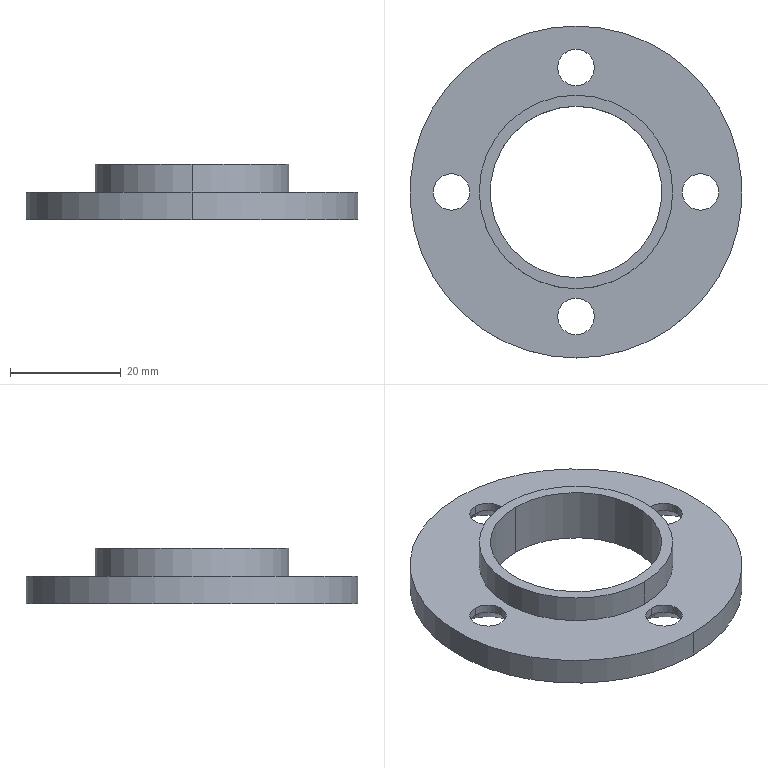Component | SolidWorks | ZDG0406-A03-P06-X1-1 | 1 solid | 25 faces | box 60 x 60 x 10 mm | volume 10063 mm3 | cylinder 14 | cone 8 | plane 3 | commonest cylinder face diameters 6.6 x8 60 x2 35 x2 31 x2 | material 45#
build123d program:
from build123d import *

# Parameters (mm, degrees)
TAPERED_COUNTERSUNK_HOLE_1_FOR_M6_HEXAGO_D           = 6.6
TAPERED_COUNTERSUNK_HOLE_1_FOR_M6_HEXAGO_CSINK_D     = 13.44
TAPERED_COUNTERSUNK_HOLE_1_FOR_M6_HEXAGO_CSINK_ANGLE = 90


with BuildPart() as part:
    # Sketch1 → Revolve1 (revolve)
    with BuildSketch(Plane.XY, mode=Mode.PRIVATE) as revolve1_sk:
        Polygon((15.5, 0), (17.5, 0), (17.5, 5), (30, 5), (30, 10), (15.5, 10), align=None)
    revolve(revolve1_sk.sketch.rotate(Axis((0, 0, 0), (0, 1, 0)), 90), axis=Axis((0, 0, 0), (0, 1, 0)))

    # Tapered Countersunk Hole 1 for M6 Hexago (through all)
    with Locations(Plane(origin=(0, 10, 0), x_dir=(1, 0, 0), z_dir=(0, 1, 0))):
        with Locations((0, 22.5), (22.5, 0), (0, -22.5), (-22.5, 0)):
            CounterSinkHole(TAPERED_COUNTERSUNK_HOLE_1_FOR_M6_HEXAGO_D / 2, TAPERED_COUNTERSUNK_HOLE_1_FOR_M6_HEXAGO_CSINK_D / 2, counter_sink_angle=TAPERED_COUNTERSUNK_HOLE_1_FOR_M6_HEXAGO_CSINK_ANGLE)


solid = part.part

# Placed as in the assembly
solid = solid.moved(Location((-22.5, 0, -15), (-90, 0, 0)))
STEP:
#1=COLOUR_RGB('',0.7922,0.8196,0.9333);
#2=FILL_AREA_STYLE_COLOUR('',#1);
#3=FILL_AREA_STYLE('',(#2));
#4=SURFACE_STYLE_FILL_AREA(#3);
#5=SURFACE_SIDE_STYLE('',(#4));
#6=SURFACE_STYLE_USAGE(.BOTH.,#5);
#7=PRESENTATION_STYLE_ASSIGNMENT((#6));
#8=CARTESIAN_POINT('',(-0.8858,-1.016,-0.8496));
#9=VERTEX_POINT('',#8);
#10=CARTESIAN_POINT('',(-0.8858,-0.7559,-0.8496));
#11=VERTEX_POINT('',#10);
#12=CARTESIAN_POINT('',(-0.8858,-0.8858,-0.8496));
#13=DIRECTION('',(0.,0.,-1.));
#14=DIRECTION('',(0.,1.,0.));
#15=AXIS2_PLACEMENT_3D('',#12,#13,#14);
#16=CIRCLE('',#15,0.1299);
#17=EDGE_CURVE('',#9,#11,#16,.T.);
#18=ORIENTED_EDGE('',*,*,#17,.F.);
#19=CARTESIAN_POINT('',(-0.8858,-1.15,-0.9843));
#20=VERTEX_POINT('',#19);
#21=CARTESIAN_POINT('',(-0.8858,-1.15,-0.9843));
#22=DIRECTION('',(0.,-0.7071,-0.7071));
#23=VECTOR('',#22,39.37);
#24=LINE('',#21,#23);
#25=EDGE_CURVE('',#9,#20,#24,.T.);
#26=ORIENTED_EDGE('',*,*,#25,.T.);
#27=CARTESIAN_POINT('',(-0.8858,-0.6213,-0.9843));
#28=VERTEX_POINT('',#27);
#29=CARTESIAN_POINT('',(-0.8858,-0.8858,-0.9843));
#30=DIRECTION('',(0.,0.,-1.));
#31=DIRECTION('',(0.,1.,0.));
#32=AXIS2_PLACEMENT_3D('',#29,#30,#31);
#33=CIRCLE('',#32,0.2646);
#34=EDGE_CURVE('',#20,#28,#33,.T.);
#35=ORIENTED_EDGE('',*,*,#34,.T.);
#36=CARTESIAN_POINT('',(-0.8858,-0.6213,-0.9843));
#37=DIRECTION('',(0.,0.7071,-0.7071));
#38=VECTOR('',#37,39.37);
#39=LINE('',#36,#38);
#40=EDGE_CURVE('',#11,#28,#39,.T.);
#41=ORIENTED_EDGE('',*,*,#40,.F.);
#42=EDGE_LOOP('',(#18,#26,#35,#41));
#43=FACE_OUTER_BOUND('',#42,.T.);
#44=CARTESIAN_POINT('',(-0.8858,-0.8858,-0.9843));
#45=DIRECTION('',(0.,0.,-1.));
#46=DIRECTION('',(0.,1.,0.));
#47=AXIS2_PLACEMENT_3D('',#44,#45,#46);
#48=CONICAL_SURFACE('',#47,0.2646,0.7854);
#49=ADVANCED_FACE('',(#43),#48,.F.);
#50=CARTESIAN_POINT('',(-0.8858,-0.7559,-0.7874));
#51=VERTEX_POINT('',#50);
#52=CARTESIAN_POINT('',(-0.8858,-1.016,-0.7874));
#53=VERTEX_POINT('',#52);
#54=CARTESIAN_POINT('',(-0.8858,-0.8858,-0.7874));
#55=DIRECTION('',(0.,0.,1.));
#56=DIRECTION('',(0.,-1.,0.));
#57=AXIS2_PLACEMENT_3D('',#54,#55,#56);
#58=CIRCLE('',#57,0.1299);
#59=EDGE_CURVE('',#51,#53,#58,.T.);
#60=ORIENTED_EDGE('',*,*,#59,.T.);
#61=CARTESIAN_POINT('',(-0.8858,-1.016,-0.9843));
#62=DIRECTION('',(0.,0.,-1.));
#63=VECTOR('',#62,39.37);
#64=LINE('',#61,#63);
#65=EDGE_CURVE('',#53,#9,#64,.T.);
#66=ORIENTED_EDGE('',*,*,#65,.T.);
#67=ORIENTED_EDGE('',*,*,#17,.T.);
#68=CARTESIAN_POINT('',(-0.8858,-0.7559,-0.9843));
#69=DIRECTION('',(0.,0.,-1.));
#70=VECTOR('',#69,39.37);
#71=LINE('',#68,#70);
#72=EDGE_CURVE('',#51,#11,#71,.T.);
#73=ORIENTED_EDGE('',*,*,#72,.F.);
#74=EDGE_LOOP('',(#60,#66,#67,#73));
#75=FACE_OUTER_BOUND('',#74,.T.);
#76=CARTESIAN_POINT('',(-0.8858,-0.8858,-0.9843));
#77=DIRECTION('',(0.,0.,-1.));
#78=DIRECTION('',(0.,1.,0.));
#79=AXIS2_PLACEMENT_3D('',#76,#77,#78);
#80=CYLINDRICAL_SURFACE('',#79,0.1299);
#81=ADVANCED_FACE('',(#75),#80,.F.);
#82=CARTESIAN_POINT('',(0.,-0.1299,-0.8496));
#83=VERTEX_POINT('',#82);
#84=CARTESIAN_POINT('',(0.,0.1299,-0.8496));
#85=VERTEX_POINT('',#84);
#86=CARTESIAN_POINT('',(0.,-0.,-0.8496));
#87=DIRECTION('',(0.,0.,-1.));
#88=DIRECTION('',(0.,1.,0.));
#89=AXIS2_PLACEMENT_3D('',#86,#87,#88);
#90=CIRCLE('',#89,0.1299);
#91=EDGE_CURVE('',#83,#85,#90,.T.);
#92=ORIENTED_EDGE('',*,*,#91,.F.);
#93=CARTESIAN_POINT('',(0.,-0.2646,-0.9843));
#94=VERTEX_POINT('',#93);
#95=CARTESIAN_POINT('',(0.,-0.2646,-0.9843));
#96=DIRECTION('',(0.,-0.7071,-0.7071));
#97=VECTOR('',#96,39.37);
#98=LINE('',#95,#97);
#99=EDGE_CURVE('',#83,#94,#98,.T.);
#100=ORIENTED_EDGE('',*,*,#99,.T.);
#101=CARTESIAN_POINT('',(0.,0.2646,-0.9843));
#102=VERTEX_POINT('',#101);
#103=CARTESIAN_POINT('',(0.,-0.,-0.9843));
#104=DIRECTION('',(0.,0.,-1.));
#105=DIRECTION('',(0.,1.,0.));
#106=AXIS2_PLACEMENT_3D('',#103,#104,#105);
#107=CIRCLE('',#106,0.2646);
#108=EDGE_CURVE('',#94,#102,#107,.T.);
#109=ORIENTED_EDGE('',*,*,#108,.T.);
#110=CARTESIAN_POINT('',(0.,0.2646,-0.9843));
#111=DIRECTION('',(0.,0.7071,-0.7071));
#112=VECTOR('',#111,39.37);
#113=LINE('',#110,#112);
#114=EDGE_CURVE('',#85,#102,#113,.T.);
#115=ORIENTED_EDGE('',*,*,#114,.F.);
#116=EDGE_LOOP('',(#92,#100,#109,#115));
#117=FACE_OUTER_BOUND('',#116,.T.);
#118=CARTESIAN_POINT('',(0.,-0.,-0.9843));
#119=DIRECTION('',(0.,0.,-1.));
#120=DIRECTION('',(0.,1.,0.));
#121=AXIS2_PLACEMENT_3D('',#118,#119,#120);
#122=CONICAL_SURFACE('',#121,0.2646,0.7854);
#123=ADVANCED_FACE('',(#117),#122,.F.);
#124=CARTESIAN_POINT('',(0.,0.1299,-0.7874));
#125=VERTEX_POINT('',#124);
#126=CARTESIAN_POINT('',(0.,-0.1299,-0.7874));
#127=VERTEX_POINT('',#126);
#128=CARTESIAN_POINT('',(0.,-0.,-0.7874));
#129=DIRECTION('',(0.,0.,1.));
#130=DIRECTION('',(0.,-1.,0.));
#131=AXIS2_PLACEMENT_3D('',#128,#129,#130);
#132=CIRCLE('',#131,0.1299);
#133=EDGE_CURVE('',#125,#127,#132,.T.);
#134=ORIENTED_EDGE('',*,*,#133,.T.);
#135=CARTESIAN_POINT('',(0.,-0.1299,-0.9843));
#136=DIRECTION('',(0.,0.,-1.));
#137=VECTOR('',#136,39.37);
#138=LINE('',#135,#137);
#139=EDGE_CURVE('',#127,#83,#138,.T.);
#140=ORIENTED_EDGE('',*,*,#139,.T.);
#141=ORIENTED_EDGE('',*,*,#91,.T.);
#142=CARTESIAN_POINT('',(0.,0.1299,-0.9843));
#143=DIRECTION('',(0.,0.,-1.));
#144=VECTOR('',#143,39.37);
#145=LINE('',#142,#144);
#146=EDGE_CURVE('',#125,#85,#145,.T.);
#147=ORIENTED_EDGE('',*,*,#146,.F.);
#148=EDGE_LOOP('',(#134,#140,#141,#147));
#149=FACE_OUTER_BOUND('',#148,.T.);
#150=CARTESIAN_POINT('',(0.,-0.,-0.9843));
#151=DIRECTION('',(0.,0.,-1.));
#152=DIRECTION('',(0.,1.,0.));
#153=AXIS2_PLACEMENT_3D('',#150,#151,#152);
#154=CYLINDRICAL_SURFACE('',#153,0.1299);
#155=ADVANCED_FACE('',(#149),#154,.F.);
#156=CARTESIAN_POINT('',(-0.8858,0.7559,-0.8496));
#157=VERTEX_POINT('',#156);
#158=CARTESIAN_POINT('',(-0.8858,1.016,-0.8496));
#159=VERTEX_POINT('',#158);
#160=CARTESIAN_POINT('',(-0.8858,0.8858,-0.8496));
#161=DIRECTION('',(0.,0.,-1.));
#162=DIRECTION('',(0.,1.,0.));
#163=AXIS2_PLACEMENT_3D('',#160,#161,#162);
#164=CIRCLE('',#163,0.1299);
#165=EDGE_CURVE('',#157,#159,#164,.T.);
#166=ORIENTED_EDGE('',*,*,#165,.F.);
#167=CARTESIAN_POINT('',(-0.8858,0.6213,-0.9843));
#168=VERTEX_POINT('',#167);
#169=CARTESIAN_POINT('',(-0.8858,0.6213,-0.9843));
#170=DIRECTION('',(0.,-0.7071,-0.7071));
#171=VECTOR('',#170,39.37);
#172=LINE('',#169,#171);
#173=EDGE_CURVE('',#157,#168,#172,.T.);
#174=ORIENTED_EDGE('',*,*,#173,.T.);
#175=CARTESIAN_POINT('',(-0.8858,1.15,-0.9843));
#176=VERTEX_POINT('',#175);
#177=CARTESIAN_POINT('',(-0.8858,0.8858,-0.9843));
#178=DIRECTION('',(0.,0.,-1.));
#179=DIRECTION('',(0.,1.,0.));
#180=AXIS2_PLACEMENT_3D('',#177,#178,#179);
#181=CIRCLE('',#180,0.2646);
#182=EDGE_CURVE('',#168,#176,#181,.T.);
#183=ORIENTED_EDGE('',*,*,#182,.T.);
#184=CARTESIAN_POINT('',(-0.8858,1.15,-0.9843));
#185=DIRECTION('',(0.,0.7071,-0.7071));
#186=VECTOR('',#185,39.37);
#187=LINE('',#184,#186);
#188=EDGE_CURVE('',#159,#176,#187,.T.);
#189=ORIENTED_EDGE('',*,*,#188,.F.);
#190=EDGE_LOOP('',(#166,#174,#183,#189));
#191=FACE_OUTER_BOUND('',#190,.T.);
#192=CARTESIAN_POINT('',(-0.8858,0.8858,-0.9843));
#193=DIRECTION('',(0.,0.,-1.));
#194=DIRECTION('',(0.,1.,0.));
#195=AXIS2_PLACEMENT_3D('',#192,#193,#194);
#196=CONICAL_SURFACE('',#195,0.2646,0.7854);
#197=ADVANCED_FACE('',(#191),#196,.F.);
#198=CARTESIAN_POINT('',(-0.8858,1.016,-0.7874));
#199=VERTEX_POINT('',#198);
#200=CARTESIAN_POINT('',(-0.8858,0.7559,-0.7874));
#201=VERTEX_POINT('',#200);
#202=CARTESIAN_POINT('',(-0.8858,0.8858,-0.7874));
#203=DIRECTION('',(0.,0.,1.));
#204=DIRECTION('',(0.,-1.,0.));
#205=AXIS2_PLACEMENT_3D('',#202,#203,#204);
#206=CIRCLE('',#205,0.1299);
#207=EDGE_CURVE('',#199,#201,#206,.T.);
#208=ORIENTED_EDGE('',*,*,#207,.T.);
#209=CARTESIAN_POINT('',(-0.8858,0.7559,-0.9843));
#210=DIRECTION('',(0.,0.,-1.));
#211=VECTOR('',#210,39.37);
#212=LINE('',#209,#211);
#213=EDGE_CURVE('',#201,#157,#212,.T.);
#214=ORIENTED_EDGE('',*,*,#213,.T.);
#215=ORIENTED_EDGE('',*,*,#165,.T.);
#216=CARTESIAN_POINT('',(-0.8858,1.016,-0.9843));
#217=DIRECTION('',(0.,0.,-1.));
#218=VECTOR('',#217,39.37);
#219=LINE('',#216,#218);
#220=EDGE_CURVE('',#199,#159,#219,.T.);
#221=ORIENTED_EDGE('',*,*,#220,.F.);
#222=EDGE_LOOP('',(#208,#214,#215,#221));
#223=FACE_OUTER_BOUND('',#222,.T.);
#224=CARTESIAN_POINT('',(-0.8858,0.8858,-0.9843));
#225=DIRECTION('',(0.,0.,-1.));
#226=DIRECTION('',(0.,1.,0.));
#227=AXIS2_PLACEMENT_3D('',#224,#225,#226);
#228=CYLINDRICAL_SURFACE('',#227,0.1299);
#229=ADVANCED_FACE('',(#223),#228,.F.);
#230=CARTESIAN_POINT('',(-1.772,-0.1299,-0.8496));
#231=VERTEX_POINT('',#230);
#232=CARTESIAN_POINT('',(-1.772,0.1299,-0.8496));
#233=VERTEX_POINT('',#232);
#234=CARTESIAN_POINT('',(-1.772,-0.,-0.8496));
#235=DIRECTION('',(0.,0.,-1.));
#236=DIRECTION('',(0.,1.,0.));
#237=AXIS2_PLACEMENT_3D('',#234,#235,#236);
#238=CIRCLE('',#237,0.1299);
#239=EDGE_CURVE('',#231,#233,#238,.T.);
#240=ORIENTED_EDGE('',*,*,#239,.F.);
#241=CARTESIAN_POINT('',(-1.772,-0.2646,-0.9843));
#242=VERTEX_POINT('',#241);
#243=CARTESIAN_POINT('',(-1.772,-0.2646,-0.9843));
#244=DIRECTION('',(0.,-0.7071,-0.7071));
#245=VECTOR('',#244,39.37);
#246=LINE('',#243,#245);
#247=EDGE_CURVE('',#231,#242,#246,.T.);
#248=ORIENTED_EDGE('',*,*,#247,.T.);
#249=CARTESIAN_POINT('',(-1.772,0.2646,-0.9843));
#250=VERTEX_POINT('',#249);
#251=CARTESIAN_POINT('',(-1.772,-0.,-0.9843));
#252=DIRECTION('',(0.,0.,-1.));
#253=DIRECTION('',(0.,1.,0.));
#254=AXIS2_PLACEMENT_3D('',#251,#252,#253);
#255=CIRCLE('',#254,0.2646);
#256=EDGE_CURVE('',#242,#250,#255,.T.);
#257=ORIENTED_EDGE('',*,*,#256,.T.);
#258=CARTESIAN_POINT('',(-1.772,0.2646,-0.9843));
#259=DIRECTION('',(0.,0.7071,-0.7071));
#260=VECTOR('',#259,39.37);
#261=LINE('',#258,#260);
#262=EDGE_CURVE('',#233,#250,#261,.T.);
#263=ORIENTED_EDGE('',*,*,#262,.F.);
#264=EDGE_LOOP('',(#240,#248,#257,#263));
#265=FACE_OUTER_BOUND('',#264,.T.);
#266=CARTESIAN_POINT('',(-1.772,-0.,-0.9843));
#267=DIRECTION('',(0.,0.,-1.));
#268=DIRECTION('',(0.,1.,0.));
#269=AXIS2_PLACEMENT_3D('',#266,#267,#268);
#270=CONICAL_SURFACE('',#269,0.2646,0.7854);
#271=ADVANCED_FACE('',(#265),#270,.F.);
#272=CARTESIAN_POINT('',(-1.772,0.1299,-0.7874));
#273=VERTEX_POINT('',#272);
#274=CARTESIAN_POINT('',(-1.772,-0.1299,-0.7874));
#275=VERTEX_POINT('',#274);
#276=CARTESIAN_POINT('',(-1.772,-0.,-0.7874));
#277=DIRECTION('',(0.,0.,1.));
#278=DIRECTION('',(0.,-1.,0.));
#279=AXIS2_PLACEMENT_3D('',#276,#277,#278);
#280=CIRCLE('',#279,0.1299);
#281=EDGE_CURVE('',#273,#275,#280,.T.);
#282=ORIENTED_EDGE('',*,*,#281,.T.);
#283=CARTESIAN_POINT('',(-1.772,-0.1299,-0.9843));
#284=DIRECTION('',(0.,0.,-1.));
#285=VECTOR('',#284,39.37);
#286=LINE('',#283,#285);
#287=EDGE_CURVE('',#275,#231,#286,.T.);
#288=ORIENTED_EDGE('',*,*,#287,.T.);
#289=ORIENTED_EDGE('',*,*,#239,.T.);
#290=CARTESIAN_POINT('',(-1.772,0.1299,-0.9843));
#291=DIRECTION('',(0.,0.,-1.));
#292=VECTOR('',#291,39.37);
#293=LINE('',#290,#292);
#294=EDGE_CURVE('',#273,#233,#293,.T.);
#295=ORIENTED_EDGE('',*,*,#294,.F.);
#296=EDGE_LOOP('',(#282,#288,#289,#295));
#297=FACE_OUTER_BOUND('',#296,.T.);
#298=CARTESIAN_POINT('',(-1.772,-0.,-0.9843));
#299=DIRECTION('',(0.,0.,-1.));
#300=DIRECTION('',(0.,1.,0.));
#301=AXIS2_PLACEMENT_3D('',#298,#299,#300);
#302=CYLINDRICAL_SURFACE('',#301,0.1299);
#303=ADVANCED_FACE('',(#297),#302,.F.);
#304=CARTESIAN_POINT('',(-0.8858,-1.181,-0.9843));
#305=VERTEX_POINT('',#304);
#306=CARTESIAN_POINT('',(-0.8858,1.181,-0.9843));
#307=VERTEX_POINT('',#306);
#308=CARTESIAN_POINT('',(-0.8858,-0.,-0.9843));
#309=DIRECTION('',(0.,0.,1.));
#310=DIRECTION('',(0.,-1.,0.));
#311=AXIS2_PLACEMENT_3D('',#308,#309,#310);
#312=CIRCLE('',#311,1.181);
#313=EDGE_CURVE('',#305,#307,#312,.T.);
#314=ORIENTED_EDGE('',*,*,#313,.T.);
#315=CARTESIAN_POINT('',(-0.8858,1.181,-0.7874));
#316=VERTEX_POINT('',#315);
#317=CARTESIAN_POINT('',(-0.8858,1.181,-0.5906));
#318=DIRECTION('',(0.,0.,1.));
#319=VECTOR('',#318,39.37);
#320=LINE('',#317,#319);
#321=EDGE_CURVE('',#307,#316,#320,.T.);
#322=ORIENTED_EDGE('',*,*,#321,.T.);
#323=CARTESIAN_POINT('',(-0.8858,-1.181,-0.7874));
#324=VERTEX_POINT('',#323);
#325=CARTESIAN_POINT('',(-0.8858,-0.,-0.7874));
#326=DIRECTION('',(0.,0.,1.));
#327=DIRECTION('',(0.,-1.,0.));
#328=AXIS2_PLACEMENT_3D('',#325,#326,#327);
#329=CIRCLE('',#328,1.181);
#330=EDGE_CURVE('',#324,#316,#329,.T.);
#331=ORIENTED_EDGE('',*,*,#330,.F.);
#332=CARTESIAN_POINT('',(-0.8858,-1.181,-0.5906));
#333=DIRECTION('',(0.,0.,1.));
#334=VECTOR('',#333,39.37);
#335=LINE('',#332,#334);
#336=EDGE_CURVE('',#305,#324,#335,.T.);
#337=ORIENTED_EDGE('',*,*,#336,.F.);
#338=EDGE_LOOP('',(#314,#322,#331,#337));
#339=FACE_OUTER_BOUND('',#338,.T.);
#340=CARTESIAN_POINT('',(-0.8858,-0.,-0.5906));
#341=DIRECTION('',(0.,0.,1.));
#342=DIRECTION('',(0.,-1.,0.));
#343=AXIS2_PLACEMENT_3D('',#340,#341,#342);
#344=CYLINDRICAL_SURFACE('',#343,1.181);
#345=ADVANCED_FACE('',(#339),#344,.T.);
#346=CARTESIAN_POINT('',(-0.8858,-0.689,-0.7874));
#347=VERTEX_POINT('',#346);
#348=CARTESIAN_POINT('',(-0.8858,0.689,-0.7874));
#349=VERTEX_POINT('',#348);
#350=CARTESIAN_POINT('',(-0.8858,-0.,-0.7874));
#351=DIRECTION('',(0.,0.,1.));
#352=DIRECTION('',(0.,-1.,0.));
#353=AXIS2_PLACEMENT_3D('',#350,#351,#352);
#354=CIRCLE('',#353,0.689);
#355=EDGE_CURVE('',#347,#349,#354,.T.);
#356=ORIENTED_EDGE('',*,*,#355,.T.);
#357=CARTESIAN_POINT('',(-0.8858,0.689,-0.5906));
#358=VERTEX_POINT('',#357);
#359=CARTESIAN_POINT('',(-0.8858,0.689,-0.5906));
#360=DIRECTION('',(0.,0.,1.));
#361=VECTOR('',#360,39.37);
#362=LINE('',#359,#361);
#363=EDGE_CURVE('',#349,#358,#362,.T.);
#364=ORIENTED_EDGE('',*,*,#363,.T.);
#365=CARTESIAN_POINT('',(-0.8858,-0.689,-0.5906));
#366=VERTEX_POINT('',#365);
#367=CARTESIAN_POINT('',(-0.8858,-0.,-0.5906));
#368=DIRECTION('',(0.,0.,1.));
#369=DIRECTION('',(0.,-1.,0.));
#370=AXIS2_PLACEMENT_3D('',#367,#368,#369);
#371=CIRCLE('',#370,0.689);
#372=EDGE_CURVE('',#366,#358,#371,.T.);
#373=ORIENTED_EDGE('',*,*,#372,.F.);
#374=CARTESIAN_POINT('',(-0.8858,-0.689,-0.5906));
#375=DIRECTION('',(0.,0.,1.));
#376=VECTOR('',#375,39.37);
#377=LINE('',#374,#376);
#378=EDGE_CURVE('',#347,#366,#377,.T.);
#379=ORIENTED_EDGE('',*,*,#378,.F.);
#380=EDGE_LOOP('',(#356,#364,#373,#379));
#381=FACE_OUTER_BOUND('',#380,.T.);
#382=CARTESIAN_POINT('',(-0.8858,-0.,-0.5906));
#383=DIRECTION('',(0.,0.,1.));
#384=DIRECTION('',(0.,-1.,0.));
#385=AXIS2_PLACEMENT_3D('',#382,#383,#384);
#386=CYLINDRICAL_SURFACE('',#385,0.689);
#387=ADVANCED_FACE('',(#381),#386,.T.);
#388=CARTESIAN_POINT('',(-0.8858,0.6102,-0.9843));
#389=VERTEX_POINT('',#388);
#390=CARTESIAN_POINT('',(-0.8858,-0.6102,-0.9843));
#391=VERTEX_POINT('',#390);
#392=CARTESIAN_POINT('',(-0.8858,-0.,-0.9843));
#393=DIRECTION('',(0.,0.,1.));
#394=DIRECTION('',(0.,-1.,0.));
#395=AXIS2_PLACEMENT_3D('',#392,#393,#394);
#396=CIRCLE('',#395,0.6102);
#397=EDGE_CURVE('',#389,#391,#396,.T.);
#398=ORIENTED_EDGE('',*,*,#397,.F.);
#399=CARTESIAN_POINT('',(-0.8858,0.6102,-0.5906));
#400=VERTEX_POINT('',#399);
#401=CARTESIAN_POINT('',(-0.8858,0.6102,-0.5906));
#402=DIRECTION('',(0.,0.,1.));
#403=VECTOR('',#402,39.37);
#404=LINE('',#401,#403);
#405=EDGE_CURVE('',#389,#400,#404,.T.);
#406=ORIENTED_EDGE('',*,*,#405,.T.);
#407=CARTESIAN_POINT('',(-0.8858,-0.6102,-0.5906));
#408=VERTEX_POINT('',#407);
#409=CARTESIAN_POINT('',(-0.8858,-0.,-0.5906));
#410=DIRECTION('',(0.,0.,1.));
#411=DIRECTION('',(0.,-1.,0.));
#412=AXIS2_PLACEMENT_3D('',#409,#410,#411);
#413=CIRCLE('',#412,0.6102);
#414=EDGE_CURVE('',#400,#408,#413,.T.);
#415=ORIENTED_EDGE('',*,*,#414,.T.);
#416=CARTESIAN_POINT('',(-0.8858,-0.6102,-0.5906));
#417=DIRECTION('',(0.,0.,1.));
#418=VECTOR('',#417,39.37);
#419=LINE('',#416,#418);
#420=EDGE_CURVE('',#391,#408,#419,.T.);
#421=ORIENTED_EDGE('',*,*,#420,.F.);
#422=EDGE_LOOP('',(#398,#406,#415,#421));
#423=FACE_OUTER_BOUND('',#422,.T.);
#424=CARTESIAN_POINT('',(-0.8858,-0.,-0.5906));
#425=DIRECTION('',(0.,0.,1.));
#426=DIRECTION('',(0.,-1.,0.));
#427=AXIS2_PLACEMENT_3D('',#424,#425,#426);
#428=CYLINDRICAL_SURFACE('',#427,0.6102);
#429=ADVANCED_FACE('',(#423),#428,.F.);
#430=ORIENTED_EDGE('',*,*,#405,.F.);
#431=CARTESIAN_POINT('',(-0.8858,-0.,-0.9843));
#432=DIRECTION('',(0.,0.,1.));
#433=DIRECTION('',(0.,-1.,0.));
#434=AXIS2_PLACEMENT_3D('',#431,#432,#433);
#435=CIRCLE('',#434,0.6102);
#436=EDGE_CURVE('',#391,#389,#435,.T.);
#437=ORIENTED_EDGE('',*,*,#436,.F.);
#438=ORIENTED_EDGE('',*,*,#420,.T.);
#439=CARTESIAN_POINT('',(-0.8858,-0.,-0.5906));
#440=DIRECTION('',(0.,0.,1.));
#441=DIRECTION('',(0.,-1.,0.));
#442=AXIS2_PLACEMENT_3D('',#439,#440,#441);
#443=CIRCLE('',#442,0.6102);
#444=EDGE_CURVE('',#408,#400,#443,.T.);
#445=ORIENTED_EDGE('',*,*,#444,.T.);
#446=EDGE_LOOP('',(#430,#437,#438,#445));
#447=FACE_OUTER_BOUND('',#446,.T.);
#448=CARTESIAN_POINT('',(-0.8858,-0.,-0.5906));
#449=DIRECTION('',(0.,0.,1.));
#450=DIRECTION('',(0.,-1.,0.));
#451=AXIS2_PLACEMENT_3D('',#448,#449,#450);
#452=CYLINDRICAL_SURFACE('',#451,0.6102);
#453=ADVANCED_FACE('',(#447),#452,.F.);
#454=ORIENTED_EDGE('',*,*,#372,.T.);
#455=CARTESIAN_POINT('',(-0.8858,-0.,-0.5906));
#456=DIRECTION('',(0.,0.,1.));
#457=DIRECTION('',(0.,-1.,0.));
#458=AXIS2_PLACEMENT_3D('',#455,#456,#457);
#459=CIRCLE('',#458,0.689);
#460=EDGE_CURVE('',#358,#366,#459,.T.);
#461=ORIENTED_EDGE('',*,*,#460,.T.);
#462=EDGE_LOOP('',(#454,#461));
#463=FACE_OUTER_BOUND('',#462,.T.);
#464=ORIENTED_EDGE('',*,*,#444,.F.);
#465=ORIENTED_EDGE('',*,*,#414,.F.);
#466=EDGE_LOOP('',(#464,#465));
#467=FACE_BOUND('',#466,.T.);
#468=CARTESIAN_POINT('',(-0.2756,-0.,-0.5906));
#469=DIRECTION('',(0.,0.,1.));
#470=DIRECTION('',(0.,-1.,0.));
#471=AXIS2_PLACEMENT_3D('',#468,#469,#470);
#472=PLANE('',#471);
#473=ADVANCED_FACE('',(#463,#467),#472,.T.);
#474=ORIENTED_EDGE('',*,*,#363,.F.);
#475=CARTESIAN_POINT('',(-0.8858,-0.,-0.7874));
#476=DIRECTION('',(0.,0.,1.));
#477=DIRECTION('',(0.,-1.,0.));
#478=AXIS2_PLACEMENT_3D('',#475,#476,#477);
#479=CIRCLE('',#478,0.689);
#480=EDGE_CURVE('',#349,#347,#479,.T.);
#481=ORIENTED_EDGE('',*,*,#480,.T.);
#482=ORIENTED_EDGE('',*,*,#378,.T.);
#483=ORIENTED_EDGE('',*,*,#460,.F.);
#484=EDGE_LOOP('',(#474,#481,#482,#483));
#485=FACE_OUTER_BOUND('',#484,.T.);
#486=CARTESIAN_POINT('',(-0.8858,-0.,-0.5906));
#487=DIRECTION('',(0.,0.,1.));
#488=DIRECTION('',(0.,-1.,0.));
#489=AXIS2_PLACEMENT_3D('',#486,#487,#488);
#490=CYLINDRICAL_SURFACE('',#489,0.689);
#491=ADVANCED_FACE('',(#485),#490,.T.);
#492=ORIENTED_EDGE('',*,*,#59,.F.);
#493=CARTESIAN_POINT('',(-0.8858,-0.8858,-0.7874));
#494=DIRECTION('',(0.,0.,1.));
#495=DIRECTION('',(0.,-1.,0.));
#496=AXIS2_PLACEMENT_3D('',#493,#494,#495);
#497=CIRCLE('',#496,0.1299);
#498=EDGE_CURVE('',#53,#51,#497,.T.);
#499=ORIENTED_EDGE('',*,*,#498,.F.);
#500=EDGE_LOOP('',(#492,#499));
#501=FACE_BOUND('',#500,.T.);
#502=ORIENTED_EDGE('',*,*,#133,.F.);
#503=CARTESIAN_POINT('',(0.,-0.,-0.7874));
#504=DIRECTION('',(0.,0.,1.));
#505=DIRECTION('',(0.,-1.,0.));
#506=AXIS2_PLACEMENT_3D('',#503,#504,#505);
#507=CIRCLE('',#506,0.1299);
#508=EDGE_CURVE('',#127,#125,#507,.T.);
#509=ORIENTED_EDGE('',*,*,#508,.F.);
#510=EDGE_LOOP('',(#502,#509));
#511=FACE_BOUND('',#510,.T.);
#512=ORIENTED_EDGE('',*,*,#207,.F.);
#513=CARTESIAN_POINT('',(-0.8858,0.8858,-0.7874));
#514=DIRECTION('',(0.,0.,1.));
#515=DIRECTION('',(0.,-1.,0.));
#516=AXIS2_PLACEMENT_3D('',#513,#514,#515);
#517=CIRCLE('',#516,0.1299);
#518=EDGE_CURVE('',#201,#199,#517,.T.);
#519=ORIENTED_EDGE('',*,*,#518,.F.);
#520=EDGE_LOOP('',(#512,#519));
#521=FACE_BOUND('',#520,.T.);
#522=ORIENTED_EDGE('',*,*,#281,.F.);
#523=CARTESIAN_POINT('',(-1.772,-0.,-0.7874));
#524=DIRECTION('',(0.,0.,1.));
#525=DIRECTION('',(0.,-1.,0.));
#526=AXIS2_PLACEMENT_3D('',#523,#524,#525);
#527=CIRCLE('',#526,0.1299);
#528=EDGE_CURVE('',#275,#273,#527,.T.);
#529=ORIENTED_EDGE('',*,*,#528,.F.);
#530=EDGE_LOOP('',(#522,#529));
#531=FACE_BOUND('',#530,.T.);
#532=ORIENTED_EDGE('',*,*,#330,.T.);
#533=CARTESIAN_POINT('',(-0.8858,-0.,-0.7874));
#534=DIRECTION('',(0.,0.,1.));
#535=DIRECTION('',(0.,-1.,0.));
#536=AXIS2_PLACEMENT_3D('',#533,#534,#535);
#537=CIRCLE('',#536,1.181);
#538=EDGE_CURVE('',#316,#324,#537,.T.);
#539=ORIENTED_EDGE('',*,*,#538,.T.);
#540=EDGE_LOOP('',(#532,#539));
#541=FACE_OUTER_BOUND('',#540,.T.);
#542=ORIENTED_EDGE('',*,*,#355,.F.);
#543=ORIENTED_EDGE('',*,*,#480,.F.);
#544=EDGE_LOOP('',(#542,#543));
#545=FACE_BOUND('',#544,.T.);
#546=CARTESIAN_POINT('',(-0.1969,-0.,-0.7874));
#547=DIRECTION('',(0.,0.,1.));
#548=DIRECTION('',(0.,-1.,0.));
#549=AXIS2_PLACEMENT_3D('',#546,#547,#548);
#550=PLANE('',#549);
#551=ADVANCED_FACE('',(#501,#511,#521,#531,#541,#545),#550,.T.);
#552=ORIENTED_EDGE('',*,*,#321,.F.);
#553=CARTESIAN_POINT('',(-0.8858,-0.,-0.9843));
#554=DIRECTION('',(0.,0.,1.));
#555=DIRECTION('',(0.,-1.,0.));
#556=AXIS2_PLACEMENT_3D('',#553,#554,#555);
#557=CIRCLE('',#556,1.181);
#558=EDGE_CURVE('',#307,#305,#557,.T.);
#559=ORIENTED_EDGE('',*,*,#558,.T.);
#560=ORIENTED_EDGE('',*,*,#336,.T.);
#561=ORIENTED_EDGE('',*,*,#538,.F.);
#562=EDGE_LOOP('',(#552,#559,#560,#561));
#563=FACE_OUTER_BOUND('',#562,.T.);
#564=CARTESIAN_POINT('',(-0.8858,-0.,-0.5906));
#565=DIRECTION('',(0.,0.,1.));
#566=DIRECTION('',(0.,-1.,0.));
#567=AXIS2_PLACEMENT_3D('',#564,#565,#566);
#568=CYLINDRICAL_SURFACE('',#567,1.181);
#569=ADVANCED_FACE('',(#563),#568,.T.);
#570=CARTESIAN_POINT('',(-0.8858,-0.8858,-0.9843));
#571=DIRECTION('',(0.,0.,-1.));
#572=DIRECTION('',(0.,1.,0.));
#573=AXIS2_PLACEMENT_3D('',#570,#571,#572);
#574=CIRCLE('',#573,0.2646);
#575=EDGE_CURVE('',#28,#20,#574,.T.);
#576=ORIENTED_EDGE('',*,*,#575,.F.);
#577=ORIENTED_EDGE('',*,*,#34,.F.);
#578=EDGE_LOOP('',(#576,#577));
#579=FACE_BOUND('',#578,.T.);
#580=CARTESIAN_POINT('',(0.,-0.,-0.9843));
#581=DIRECTION('',(0.,0.,-1.));
#582=DIRECTION('',(0.,1.,0.));
#583=AXIS2_PLACEMENT_3D('',#580,#581,#582);
#584=CIRCLE('',#583,0.2646);
#585=EDGE_CURVE('',#102,#94,#584,.T.);
#586=ORIENTED_EDGE('',*,*,#585,.F.);
#587=ORIENTED_EDGE('',*,*,#108,.F.);
#588=EDGE_LOOP('',(#586,#587));
#589=FACE_BOUND('',#588,.T.);
#590=CARTESIAN_POINT('',(-0.8858,0.8858,-0.9843));
#591=DIRECTION('',(0.,0.,-1.));
#592=DIRECTION('',(0.,1.,0.));
#593=AXIS2_PLACEMENT_3D('',#590,#591,#592);
#594=CIRCLE('',#593,0.2646);
#595=EDGE_CURVE('',#176,#168,#594,.T.);
#596=ORIENTED_EDGE('',*,*,#595,.F.);
#597=ORIENTED_EDGE('',*,*,#182,.F.);
#598=EDGE_LOOP('',(#596,#597));
#599=FACE_BOUND('',#598,.T.);
#600=CARTESIAN_POINT('',(-1.772,-0.,-0.9843));
#601=DIRECTION('',(0.,0.,-1.));
#602=DIRECTION('',(0.,1.,0.));
#603=AXIS2_PLACEMENT_3D('',#600,#601,#602);
#604=CIRCLE('',#603,0.2646);
#605=EDGE_CURVE('',#250,#242,#604,.T.);
#606=ORIENTED_EDGE('',*,*,#605,.F.);
#607=ORIENTED_EDGE('',*,*,#256,.F.);
#608=EDGE_LOOP('',(#606,#607));
#609=FACE_BOUND('',#608,.T.);
#610=ORIENTED_EDGE('',*,*,#436,.T.);
#611=ORIENTED_EDGE('',*,*,#397,.T.);
#612=EDGE_LOOP('',(#610,#611));
#613=FACE_BOUND('',#612,.T.);
#614=ORIENTED_EDGE('',*,*,#313,.F.);
#615=ORIENTED_EDGE('',*,*,#558,.F.);
#616=EDGE_LOOP('',(#614,#615));
#617=FACE_OUTER_BOUND('',#616,.T.);
#618=CARTESIAN_POINT('',(0.2953,-0.,-0.9843));
#619=DIRECTION('',(0.,0.,-1.));
#620=DIRECTION('',(0.,1.,0.));
#621=AXIS2_PLACEMENT_3D('',#618,#619,#620);
#622=PLANE('',#621);
#623=ADVANCED_FACE('',(#579,#589,#599,#609,#613,#617),#622,.T.);
#624=ORIENTED_EDGE('',*,*,#287,.F.);
#625=ORIENTED_EDGE('',*,*,#528,.T.);
#626=ORIENTED_EDGE('',*,*,#294,.T.);
#627=CARTESIAN_POINT('',(-1.772,-0.,-0.8496));
#628=DIRECTION('',(0.,0.,-1.));
#629=DIRECTION('',(0.,1.,0.));
#630=AXIS2_PLACEMENT_3D('',#627,#628,#629);
#631=CIRCLE('',#630,0.1299);
#632=EDGE_CURVE('',#233,#231,#631,.T.);
#633=ORIENTED_EDGE('',*,*,#632,.T.);
#634=EDGE_LOOP('',(#624,#625,#626,#633));
#635=FACE_OUTER_BOUND('',#634,.T.);
#636=CARTESIAN_POINT('',(-1.772,-0.,-0.9843));
#637=DIRECTION('',(0.,0.,-1.));
#638=DIRECTION('',(0.,1.,0.));
#639=AXIS2_PLACEMENT_3D('',#636,#637,#638);
#640=CYLINDRICAL_SURFACE('',#639,0.1299);
#641=ADVANCED_FACE('',(#635),#640,.F.);
#642=ORIENTED_EDGE('',*,*,#247,.F.);
#643=ORIENTED_EDGE('',*,*,#632,.F.);
#644=ORIENTED_EDGE('',*,*,#262,.T.);
#645=ORIENTED_EDGE('',*,*,#605,.T.);
#646=EDGE_LOOP('',(#642,#643,#644,#645));
#647=FACE_OUTER_BOUND('',#646,.T.);
#648=CARTESIAN_POINT('',(-1.772,-0.,-0.9843));
#649=DIRECTION('',(0.,0.,-1.));
#650=DIRECTION('',(0.,1.,0.));
#651=AXIS2_PLACEMENT_3D('',#648,#649,#650);
#652=CONICAL_SURFACE('',#651,0.2646,0.7854);
#653=ADVANCED_FACE('',(#647),#652,.F.);
#654=ORIENTED_EDGE('',*,*,#213,.F.);
#655=ORIENTED_EDGE('',*,*,#518,.T.);
#656=ORIENTED_EDGE('',*,*,#220,.T.);
#657=CARTESIAN_POINT('',(-0.8858,0.8858,-0.8496));
#658=DIRECTION('',(0.,0.,-1.));
#659=DIRECTION('',(0.,1.,0.));
#660=AXIS2_PLACEMENT_3D('',#657,#658,#659);
#661=CIRCLE('',#660,0.1299);
#662=EDGE_CURVE('',#159,#157,#661,.T.);
#663=ORIENTED_EDGE('',*,*,#662,.T.);
#664=EDGE_LOOP('',(#654,#655,#656,#663));
#665=FACE_OUTER_BOUND('',#664,.T.);
#666=CARTESIAN_POINT('',(-0.8858,0.8858,-0.9843));
#667=DIRECTION('',(0.,0.,-1.));
#668=DIRECTION('',(0.,1.,0.));
#669=AXIS2_PLACEMENT_3D('',#666,#667,#668);
#670=CYLINDRICAL_SURFACE('',#669,0.1299);
#671=ADVANCED_FACE('',(#665),#670,.F.);
#672=ORIENTED_EDGE('',*,*,#173,.F.);
#673=ORIENTED_EDGE('',*,*,#662,.F.);
#674=ORIENTED_EDGE('',*,*,#188,.T.);
#675=ORIENTED_EDGE('',*,*,#595,.T.);
#676=EDGE_LOOP('',(#672,#673,#674,#675));
#677=FACE_OUTER_BOUND('',#676,.T.);
#678=CARTESIAN_POINT('',(-0.8858,0.8858,-0.9843));
#679=DIRECTION('',(0.,0.,-1.));
#680=DIRECTION('',(0.,1.,0.));
#681=AXIS2_PLACEMENT_3D('',#678,#679,#680);
#682=CONICAL_SURFACE('',#681,0.2646,0.7854);
#683=ADVANCED_FACE('',(#677),#682,.F.);
#684=ORIENTED_EDGE('',*,*,#139,.F.);
#685=ORIENTED_EDGE('',*,*,#508,.T.);
#686=ORIENTED_EDGE('',*,*,#146,.T.);
#687=CARTESIAN_POINT('',(0.,-0.,-0.8496));
#688=DIRECTION('',(0.,0.,-1.));
#689=DIRECTION('',(0.,1.,0.));
#690=AXIS2_PLACEMENT_3D('',#687,#688,#689);
#691=CIRCLE('',#690,0.1299);
#692=EDGE_CURVE('',#85,#83,#691,.T.);
#693=ORIENTED_EDGE('',*,*,#692,.T.);
#694=EDGE_LOOP('',(#684,#685,#686,#693));
#695=FACE_OUTER_BOUND('',#694,.T.);
#696=CARTESIAN_POINT('',(0.,-0.,-0.9843));
#697=DIRECTION('',(0.,0.,-1.));
#698=DIRECTION('',(0.,1.,0.));
#699=AXIS2_PLACEMENT_3D('',#696,#697,#698);
#700=CYLINDRICAL_SURFACE('',#699,0.1299);
#701=ADVANCED_FACE('',(#695),#700,.F.);
#702=ORIENTED_EDGE('',*,*,#99,.F.);
#703=ORIENTED_EDGE('',*,*,#692,.F.);
#704=ORIENTED_EDGE('',*,*,#114,.T.);
#705=ORIENTED_EDGE('',*,*,#585,.T.);
#706=EDGE_LOOP('',(#702,#703,#704,#705));
#707=FACE_OUTER_BOUND('',#706,.T.);
#708=CARTESIAN_POINT('',(0.,-0.,-0.9843));
#709=DIRECTION('',(0.,0.,-1.));
#710=DIRECTION('',(0.,1.,0.));
#711=AXIS2_PLACEMENT_3D('',#708,#709,#710);
#712=CONICAL_SURFACE('',#711,0.2646,0.7854);
#713=ADVANCED_FACE('',(#707),#712,.F.);
#714=ORIENTED_EDGE('',*,*,#65,.F.);
#715=ORIENTED_EDGE('',*,*,#498,.T.);
#716=ORIENTED_EDGE('',*,*,#72,.T.);
#717=CARTESIAN_POINT('',(-0.8858,-0.8858,-0.8496));
#718=DIRECTION('',(0.,0.,-1.));
#719=DIRECTION('',(0.,1.,0.));
#720=AXIS2_PLACEMENT_3D('',#717,#718,#719);
#721=CIRCLE('',#720,0.1299);
#722=EDGE_CURVE('',#11,#9,#721,.T.);
#723=ORIENTED_EDGE('',*,*,#722,.T.);
#724=EDGE_LOOP('',(#714,#715,#716,#723));
#725=FACE_OUTER_BOUND('',#724,.T.);
#726=CARTESIAN_POINT('',(-0.8858,-0.8858,-0.9843));
#727=DIRECTION('',(0.,0.,-1.));
#728=DIRECTION('',(0.,1.,0.));
#729=AXIS2_PLACEMENT_3D('',#726,#727,#728);
#730=CYLINDRICAL_SURFACE('',#729,0.1299);
#731=ADVANCED_FACE('',(#725),#730,.F.);
#732=ORIENTED_EDGE('',*,*,#25,.F.);
#733=ORIENTED_EDGE('',*,*,#722,.F.);
#734=ORIENTED_EDGE('',*,*,#40,.T.);
#735=ORIENTED_EDGE('',*,*,#575,.T.);
#736=EDGE_LOOP('',(#732,#733,#734,#735));
#737=FACE_OUTER_BOUND('',#736,.T.);
#738=CARTESIAN_POINT('',(-0.8858,-0.8858,-0.9843));
#739=DIRECTION('',(0.,0.,-1.));
#740=DIRECTION('',(0.,1.,0.));
#741=AXIS2_PLACEMENT_3D('',#738,#739,#740);
#742=CONICAL_SURFACE('',#741,0.2646,0.7854);
#743=ADVANCED_FACE('',(#737),#742,.F.);
#744=CLOSED_SHELL('',(#49,#81,#123,#155,#197,#229,#271,#303,#345,#387,#429,#453,#473,#491,#551,#569,#623,#641,#653,#671,#683,#701,#713,#731,#743));
#745=MANIFOLD_SOLID_BREP('',#744);
#746=STYLED_ITEM('',(#7),#745);
#747=PRESENTATION_LAYER_ASSIGNMENT('','',(#746));
#748=(LENGTH_UNIT()NAMED_UNIT(*)SI_UNIT($,.METRE.));
#749=LENGTH_MEASURE_WITH_UNIT(LENGTH_MEASURE(0.0254),#748);
#750=DIMENSIONAL_EXPONENTS(1.,0.,0.,0.,0.,0.,0.);
#751=(CONVERSION_BASED_UNIT('',#749)LENGTH_UNIT()NAMED_UNIT(#750));
#752=UNCERTAINTY_MEASURE_WITH_UNIT(LENGTH_MEASURE(0.00001),#751,'','');
#753=(NAMED_UNIT(*)PLANE_ANGLE_UNIT()SI_UNIT($,.RADIAN.));
#754=(NAMED_UNIT(*)SI_UNIT($,.STERADIAN.)SOLID_ANGLE_UNIT());
#755=(GEOMETRIC_REPRESENTATION_CONTEXT(3)GLOBAL_UNCERTAINTY_ASSIGNED_CONTEXT((#752))GLOBAL_UNIT_ASSIGNED_CONTEXT((#751,#753,#754))REPRESENTATION_CONTEXT('',''));
#756=MECHANICAL_DESIGN_GEOMETRIC_PRESENTATION_REPRESENTATION('',(#746),#755);
#757=CARTESIAN_POINT('',(0.,0.,0.));
#758=DIRECTION('',(0.,0.,1.));
#759=DIRECTION('',(1.,0.,0.));
#760=AXIS2_PLACEMENT_3D('',#757,#758,#759);
#761=(LENGTH_UNIT()NAMED_UNIT(*)SI_UNIT($,.METRE.));
#762=LENGTH_MEASURE_WITH_UNIT(LENGTH_MEASURE(0.0254),#761);
#763=DIMENSIONAL_EXPONENTS(1.,0.,0.,0.,0.,0.,0.);
#764=(CONVERSION_BASED_UNIT('',#762)LENGTH_UNIT()NAMED_UNIT(#763));
#765=UNCERTAINTY_MEASURE_WITH_UNIT(LENGTH_MEASURE(0.00001),#764,'','');
#766=(NAMED_UNIT(*)PLANE_ANGLE_UNIT()SI_UNIT($,.RADIAN.));
#767=(NAMED_UNIT(*)SI_UNIT($,.STERADIAN.)SOLID_ANGLE_UNIT());
#768=(GEOMETRIC_REPRESENTATION_CONTEXT(3)GLOBAL_UNCERTAINTY_ASSIGNED_CONTEXT((#765))GLOBAL_UNIT_ASSIGNED_CONTEXT((#764,#766,#767))REPRESENTATION_CONTEXT('',''));
#769=ADVANCED_BREP_SHAPE_REPRESENTATION('',(#745,#760),#768);